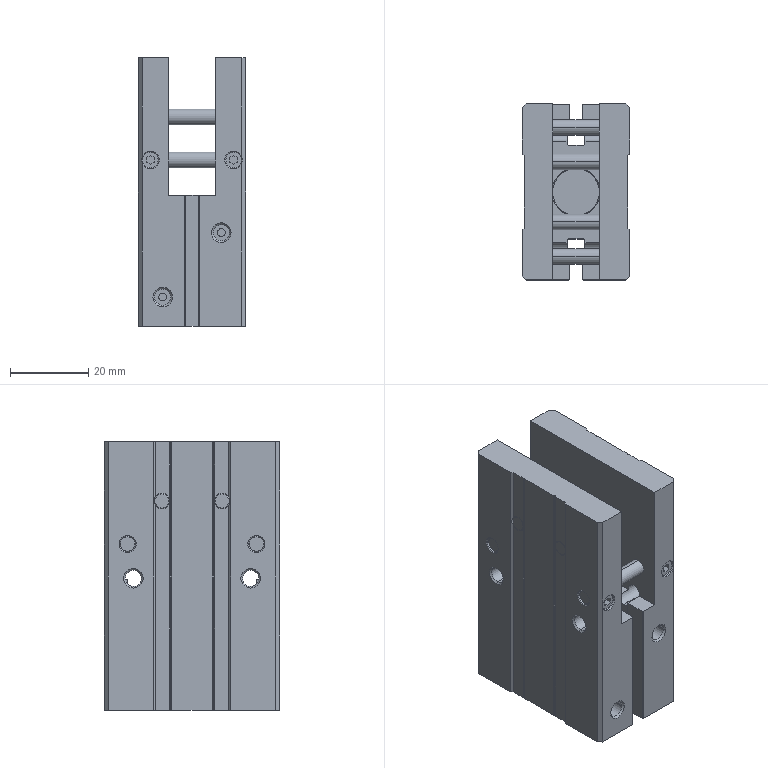Component | SolidWorks | HZ022-HFP20-1_HZ022-HFP20 (2)-1 | 1 solid | 257 faces | volume 54250 mm3 | plane 121 | cylinder 80 | cone 56 | commonest cylinder face diameters 4 x32 4.134 x20 0.4 x12 2 x4 0.8 x4 12 x2 21 x2 20 x2 | material AL6061